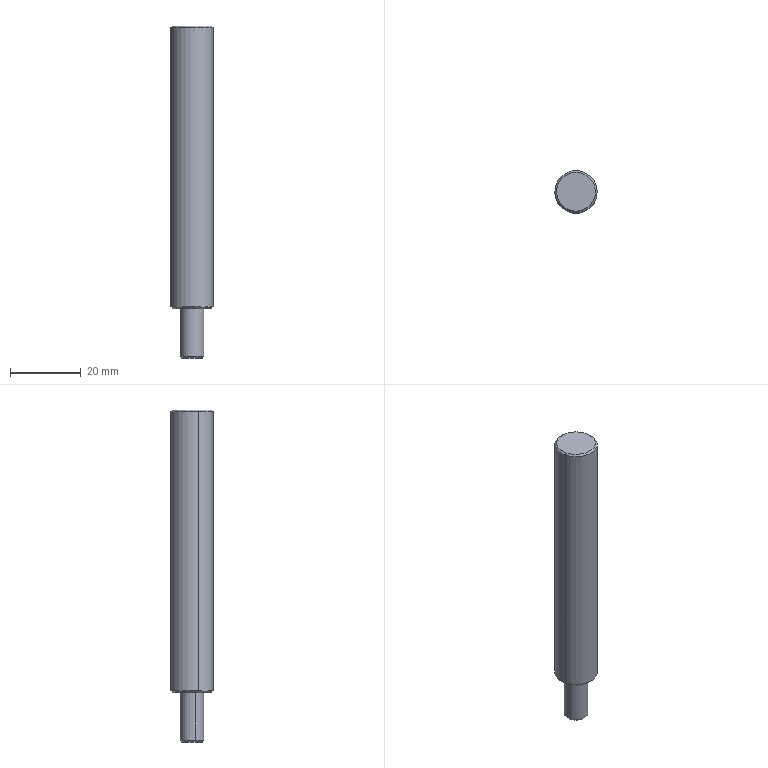Component | SolidWorks | GuidePost-2 | 1 solid | 13 faces | box 12 x 12 x 94 mm | volume 9545 mm3 | cone 6 | cylinder 4 | plane 3 | commonest cylinder face diameters 6.8 x2 12 x2
build123d program:
from build123d import *


with BuildPart() as part:
    # Sketch1 → Revolve1 (revolve)
    with BuildSketch(Plane.XY, mode=Mode.PRIVATE) as revolve1_sk:
        Polygon((0, 5.5), (0, 0), (94, 0), (94, 2.9), (93.5, 3.4), (80, 3.4), (80, 5.5), (79.5, 6), (0.5, 6), align=None)
    revolve(revolve1_sk.sketch.rotate(Axis((0, 0, 0), (1, 0, 0)), 270), axis=Axis((0, 0, 0), (1, 0, 0)))


solid = part.part

# Placed as in the assembly
solid = solid.moved(Location((0, -65, 350.554), (0, 90, 0)))
STEP:
#1=COLOUR_RGB('',0.7922,0.8196,0.9333);
#2=FILL_AREA_STYLE_COLOUR('',#1);
#3=FILL_AREA_STYLE('',(#2));
#4=SURFACE_STYLE_FILL_AREA(#3);
#5=SURFACE_SIDE_STYLE('',(#4));
#6=SURFACE_STYLE_USAGE(.BOTH.,#5);
#7=PRESENTATION_STYLE_ASSIGNMENT((#6));
#8=CARTESIAN_POINT('',(-0.109,-2.593,10.101));
#9=VERTEX_POINT('',#8);
#10=CARTESIAN_POINT('',(0.109,-2.525,10.101));
#11=VERTEX_POINT('',#10);
#12=CARTESIAN_POINT('',(-0.,-2.559,10.101));
#13=DIRECTION('',(0.,0.,-1.));
#14=DIRECTION('',(-0.9544,-0.2985,0.));
#15=AXIS2_PLACEMENT_3D('',#12,#13,#14);
#16=CIRCLE('',#15,0.1142);
#17=EDGE_CURVE('',#9,#11,#16,.T.);
#18=ORIENTED_EDGE('',*,*,#17,.F.);
#19=CARTESIAN_POINT('',(-0.1278,-2.599,10.12));
#20=VERTEX_POINT('',#19);
#21=CARTESIAN_POINT('',(-0.109,-2.593,10.101));
#22=DIRECTION('',(-0.6749,-0.2111,0.7071));
#23=VECTOR('',#22,39.37);
#24=LINE('',#21,#23);
#25=EDGE_CURVE('',#9,#20,#24,.T.);
#26=ORIENTED_EDGE('',*,*,#25,.T.);
#27=CARTESIAN_POINT('',(0.1278,-2.519,10.12));
#28=VERTEX_POINT('',#27);
#29=CARTESIAN_POINT('',(-0.,-2.559,10.12));
#30=DIRECTION('',(0.,0.,-1.));
#31=DIRECTION('',(-0.9544,-0.2985,0.));
#32=AXIS2_PLACEMENT_3D('',#29,#30,#31);
#33=CIRCLE('',#32,0.1339);
#34=EDGE_CURVE('',#20,#28,#33,.T.);
#35=ORIENTED_EDGE('',*,*,#34,.T.);
#36=CARTESIAN_POINT('',(0.109,-2.525,10.101));
#37=DIRECTION('',(0.6749,0.2111,0.7071));
#38=VECTOR('',#37,39.37);
#39=LINE('',#36,#38);
#40=EDGE_CURVE('',#11,#28,#39,.T.);
#41=ORIENTED_EDGE('',*,*,#40,.F.);
#42=EDGE_LOOP('',(#18,#26,#35,#41));
#43=FACE_OUTER_BOUND('',#42,.T.);
#44=CARTESIAN_POINT('',(-0.,-2.559,10.101));
#45=DIRECTION('',(-0.,-0.,1.));
#46=DIRECTION('',(0.9544,0.2985,0.));
#47=AXIS2_PLACEMENT_3D('',#44,#45,#46);
#48=CONICAL_SURFACE('',#47,0.1142,0.7854);
#49=ADVANCED_FACE('',(#43),#48,.T.);
#50=CARTESIAN_POINT('',(-0.1278,-2.599,10.652));
#51=VERTEX_POINT('',#50);
#52=CARTESIAN_POINT('',(0.1278,-2.519,10.652));
#53=VERTEX_POINT('',#52);
#54=CARTESIAN_POINT('',(-0.,-2.559,10.652));
#55=DIRECTION('',(0.,0.,-1.));
#56=DIRECTION('',(-0.9544,-0.2985,0.));
#57=AXIS2_PLACEMENT_3D('',#54,#55,#56);
#58=CIRCLE('',#57,0.1339);
#59=EDGE_CURVE('',#51,#53,#58,.T.);
#60=ORIENTED_EDGE('',*,*,#59,.T.);
#61=CARTESIAN_POINT('',(0.1278,-2.519,13.801));
#62=DIRECTION('',(0.,0.,-1.));
#63=VECTOR('',#62,39.37);
#64=LINE('',#61,#63);
#65=EDGE_CURVE('',#53,#28,#64,.T.);
#66=ORIENTED_EDGE('',*,*,#65,.T.);
#67=ORIENTED_EDGE('',*,*,#34,.F.);
#68=CARTESIAN_POINT('',(-0.1278,-2.599,13.801));
#69=DIRECTION('',(0.,0.,-1.));
#70=VECTOR('',#69,39.37);
#71=LINE('',#68,#70);
#72=EDGE_CURVE('',#51,#20,#71,.T.);
#73=ORIENTED_EDGE('',*,*,#72,.F.);
#74=EDGE_LOOP('',(#60,#66,#67,#73));
#75=FACE_OUTER_BOUND('',#74,.T.);
#76=CARTESIAN_POINT('',(-0.,-2.559,13.801));
#77=DIRECTION('',(0.,0.,-1.));
#78=DIRECTION('',(-0.9544,-0.2985,0.));
#79=AXIS2_PLACEMENT_3D('',#76,#77,#78);
#80=CYLINDRICAL_SURFACE('',#79,0.1339);
#81=ADVANCED_FACE('',(#75),#80,.T.);
#82=CARTESIAN_POINT('',(-0.2067,-2.624,10.652));
#83=VERTEX_POINT('',#82);
#84=CARTESIAN_POINT('',(0.2067,-2.494,10.652));
#85=VERTEX_POINT('',#84);
#86=CARTESIAN_POINT('',(-0.,-2.559,10.652));
#87=DIRECTION('',(0.,0.,-1.));
#88=DIRECTION('',(-0.9544,-0.2985,0.));
#89=AXIS2_PLACEMENT_3D('',#86,#87,#88);
#90=CIRCLE('',#89,0.2165);
#91=EDGE_CURVE('',#83,#85,#90,.T.);
#92=ORIENTED_EDGE('',*,*,#91,.F.);
#93=CARTESIAN_POINT('',(-0.2255,-2.63,10.671));
#94=VERTEX_POINT('',#93);
#95=CARTESIAN_POINT('',(-0.2067,-2.624,10.652));
#96=DIRECTION('',(-0.6749,-0.2111,0.7071));
#97=VECTOR('',#96,39.37);
#98=LINE('',#95,#97);
#99=EDGE_CURVE('',#83,#94,#98,.T.);
#100=ORIENTED_EDGE('',*,*,#99,.T.);
#101=CARTESIAN_POINT('',(0.2255,-2.489,10.671));
#102=VERTEX_POINT('',#101);
#103=CARTESIAN_POINT('',(-0.,-2.559,10.671));
#104=DIRECTION('',(0.,0.,-1.));
#105=DIRECTION('',(-0.9544,-0.2985,0.));
#106=AXIS2_PLACEMENT_3D('',#103,#104,#105);
#107=CIRCLE('',#106,0.2362);
#108=EDGE_CURVE('',#94,#102,#107,.T.);
#109=ORIENTED_EDGE('',*,*,#108,.T.);
#110=CARTESIAN_POINT('',(0.2067,-2.494,10.652));
#111=DIRECTION('',(0.6749,0.2111,0.7071));
#112=VECTOR('',#111,39.37);
#113=LINE('',#110,#112);
#114=EDGE_CURVE('',#85,#102,#113,.T.);
#115=ORIENTED_EDGE('',*,*,#114,.F.);
#116=EDGE_LOOP('',(#92,#100,#109,#115));
#117=FACE_OUTER_BOUND('',#116,.T.);
#118=CARTESIAN_POINT('',(-0.,-2.559,10.652));
#119=DIRECTION('',(-0.,-0.,1.));
#120=DIRECTION('',(0.9544,0.2985,0.));
#121=AXIS2_PLACEMENT_3D('',#118,#119,#120);
#122=CONICAL_SURFACE('',#121,0.2165,0.7854);
#123=ADVANCED_FACE('',(#117),#122,.T.);
#124=CARTESIAN_POINT('',(-0.2255,-2.63,13.782));
#125=VERTEX_POINT('',#124);
#126=CARTESIAN_POINT('',(0.2255,-2.489,13.782));
#127=VERTEX_POINT('',#126);
#128=CARTESIAN_POINT('',(-0.,-2.559,13.782));
#129=DIRECTION('',(0.,0.,-1.));
#130=DIRECTION('',(-0.9544,-0.2985,0.));
#131=AXIS2_PLACEMENT_3D('',#128,#129,#130);
#132=CIRCLE('',#131,0.2362);
#133=EDGE_CURVE('',#125,#127,#132,.T.);
#134=ORIENTED_EDGE('',*,*,#133,.T.);
#135=CARTESIAN_POINT('',(0.2255,-2.489,13.801));
#136=DIRECTION('',(0.,0.,-1.));
#137=VECTOR('',#136,39.37);
#138=LINE('',#135,#137);
#139=EDGE_CURVE('',#127,#102,#138,.T.);
#140=ORIENTED_EDGE('',*,*,#139,.T.);
#141=ORIENTED_EDGE('',*,*,#108,.F.);
#142=CARTESIAN_POINT('',(-0.2255,-2.63,13.801));
#143=DIRECTION('',(0.,0.,-1.));
#144=VECTOR('',#143,39.37);
#145=LINE('',#142,#144);
#146=EDGE_CURVE('',#125,#94,#145,.T.);
#147=ORIENTED_EDGE('',*,*,#146,.F.);
#148=EDGE_LOOP('',(#134,#140,#141,#147));
#149=FACE_OUTER_BOUND('',#148,.T.);
#150=CARTESIAN_POINT('',(-0.,-2.559,13.801));
#151=DIRECTION('',(0.,0.,-1.));
#152=DIRECTION('',(-0.9544,-0.2985,0.));
#153=AXIS2_PLACEMENT_3D('',#150,#151,#152);
#154=CYLINDRICAL_SURFACE('',#153,0.2362);
#155=ADVANCED_FACE('',(#149),#154,.T.);
#156=CARTESIAN_POINT('',(-0.2067,-2.624,13.801));
#157=VERTEX_POINT('',#156);
#158=CARTESIAN_POINT('',(0.2067,-2.494,13.801));
#159=VERTEX_POINT('',#158);
#160=CARTESIAN_POINT('',(-0.,-2.559,13.801));
#161=DIRECTION('',(0.,0.,-1.));
#162=DIRECTION('',(-0.9544,-0.2985,0.));
#163=AXIS2_PLACEMENT_3D('',#160,#161,#162);
#164=CIRCLE('',#163,0.2165);
#165=EDGE_CURVE('',#157,#159,#164,.T.);
#166=ORIENTED_EDGE('',*,*,#165,.T.);
#167=CARTESIAN_POINT('',(0.2255,-2.489,13.782));
#168=DIRECTION('',(0.6749,0.2111,-0.7071));
#169=VECTOR('',#168,39.37);
#170=LINE('',#167,#169);
#171=EDGE_CURVE('',#159,#127,#170,.T.);
#172=ORIENTED_EDGE('',*,*,#171,.T.);
#173=ORIENTED_EDGE('',*,*,#133,.F.);
#174=CARTESIAN_POINT('',(-0.2255,-2.63,13.782));
#175=DIRECTION('',(-0.6749,-0.2111,-0.7071));
#176=VECTOR('',#175,39.37);
#177=LINE('',#174,#176);
#178=EDGE_CURVE('',#157,#125,#177,.T.);
#179=ORIENTED_EDGE('',*,*,#178,.F.);
#180=EDGE_LOOP('',(#166,#172,#173,#179));
#181=FACE_OUTER_BOUND('',#180,.T.);
#182=CARTESIAN_POINT('',(-0.,-2.559,13.782));
#183=DIRECTION('',(0.,0.,-1.));
#184=DIRECTION('',(-0.9544,-0.2985,0.));
#185=AXIS2_PLACEMENT_3D('',#182,#183,#184);
#186=CONICAL_SURFACE('',#185,0.2362,0.7854);
#187=ADVANCED_FACE('',(#181),#186,.T.);
#188=ORIENTED_EDGE('',*,*,#171,.F.);
#189=CARTESIAN_POINT('',(-0.,-2.559,13.801));
#190=DIRECTION('',(0.,0.,-1.));
#191=DIRECTION('',(-0.9544,-0.2985,0.));
#192=AXIS2_PLACEMENT_3D('',#189,#190,#191);
#193=CIRCLE('',#192,0.2165);
#194=EDGE_CURVE('',#159,#157,#193,.T.);
#195=ORIENTED_EDGE('',*,*,#194,.T.);
#196=ORIENTED_EDGE('',*,*,#178,.T.);
#197=CARTESIAN_POINT('',(-0.,-2.559,13.782));
#198=DIRECTION('',(0.,0.,-1.));
#199=DIRECTION('',(-0.9544,-0.2985,0.));
#200=AXIS2_PLACEMENT_3D('',#197,#198,#199);
#201=CIRCLE('',#200,0.2362);
#202=EDGE_CURVE('',#127,#125,#201,.T.);
#203=ORIENTED_EDGE('',*,*,#202,.F.);
#204=EDGE_LOOP('',(#188,#195,#196,#203));
#205=FACE_OUTER_BOUND('',#204,.T.);
#206=CARTESIAN_POINT('',(-0.,-2.559,13.782));
#207=DIRECTION('',(0.,0.,-1.));
#208=DIRECTION('',(-0.9544,-0.2985,0.));
#209=AXIS2_PLACEMENT_3D('',#206,#207,#208);
#210=CONICAL_SURFACE('',#209,0.2362,0.7854);
#211=ADVANCED_FACE('',(#205),#210,.T.);
#212=ORIENTED_EDGE('',*,*,#139,.F.);
#213=ORIENTED_EDGE('',*,*,#202,.T.);
#214=ORIENTED_EDGE('',*,*,#146,.T.);
#215=CARTESIAN_POINT('',(-0.,-2.559,10.671));
#216=DIRECTION('',(0.,0.,-1.));
#217=DIRECTION('',(-0.9544,-0.2985,0.));
#218=AXIS2_PLACEMENT_3D('',#215,#216,#217);
#219=CIRCLE('',#218,0.2362);
#220=EDGE_CURVE('',#102,#94,#219,.T.);
#221=ORIENTED_EDGE('',*,*,#220,.F.);
#222=EDGE_LOOP('',(#212,#213,#214,#221));
#223=FACE_OUTER_BOUND('',#222,.T.);
#224=CARTESIAN_POINT('',(-0.,-2.559,13.801));
#225=DIRECTION('',(0.,0.,-1.));
#226=DIRECTION('',(-0.9544,-0.2985,0.));
#227=AXIS2_PLACEMENT_3D('',#224,#225,#226);
#228=CYLINDRICAL_SURFACE('',#227,0.2362);
#229=ADVANCED_FACE('',(#223),#228,.T.);
#230=ORIENTED_EDGE('',*,*,#99,.F.);
#231=CARTESIAN_POINT('',(-0.,-2.559,10.652));
#232=DIRECTION('',(0.,0.,-1.));
#233=DIRECTION('',(-0.9544,-0.2985,0.));
#234=AXIS2_PLACEMENT_3D('',#231,#232,#233);
#235=CIRCLE('',#234,0.2165);
#236=EDGE_CURVE('',#85,#83,#235,.T.);
#237=ORIENTED_EDGE('',*,*,#236,.F.);
#238=ORIENTED_EDGE('',*,*,#114,.T.);
#239=ORIENTED_EDGE('',*,*,#220,.T.);
#240=EDGE_LOOP('',(#230,#237,#238,#239));
#241=FACE_OUTER_BOUND('',#240,.T.);
#242=CARTESIAN_POINT('',(-0.,-2.559,10.652));
#243=DIRECTION('',(-0.,-0.,1.));
#244=DIRECTION('',(0.9544,0.2985,0.));
#245=AXIS2_PLACEMENT_3D('',#242,#243,#244);
#246=CONICAL_SURFACE('',#245,0.2165,0.7854);
#247=ADVANCED_FACE('',(#241),#246,.T.);
#248=ORIENTED_EDGE('',*,*,#236,.T.);
#249=ORIENTED_EDGE('',*,*,#91,.T.);
#250=EDGE_LOOP('',(#248,#249));
#251=FACE_OUTER_BOUND('',#250,.T.);
#252=ORIENTED_EDGE('',*,*,#59,.F.);
#253=CARTESIAN_POINT('',(-0.,-2.559,10.652));
#254=DIRECTION('',(0.,0.,-1.));
#255=DIRECTION('',(-0.9544,-0.2985,0.));
#256=AXIS2_PLACEMENT_3D('',#253,#254,#255);
#257=CIRCLE('',#256,0.1339);
#258=EDGE_CURVE('',#53,#51,#257,.T.);
#259=ORIENTED_EDGE('',*,*,#258,.F.);
#260=EDGE_LOOP('',(#252,#259));
#261=FACE_BOUND('',#260,.T.);
#262=CARTESIAN_POINT('',(-0.03995,-2.431,10.652));
#263=DIRECTION('',(0.,0.,-1.));
#264=DIRECTION('',(-0.9544,-0.2985,-0.));
#265=AXIS2_PLACEMENT_3D('',#262,#263,#264);
#266=PLANE('',#265);
#267=ADVANCED_FACE('',(#251,#261),#266,.T.);
#268=ORIENTED_EDGE('',*,*,#65,.F.);
#269=ORIENTED_EDGE('',*,*,#258,.T.);
#270=ORIENTED_EDGE('',*,*,#72,.T.);
#271=CARTESIAN_POINT('',(-0.,-2.559,10.12));
#272=DIRECTION('',(0.,0.,-1.));
#273=DIRECTION('',(-0.9544,-0.2985,0.));
#274=AXIS2_PLACEMENT_3D('',#271,#272,#273);
#275=CIRCLE('',#274,0.1339);
#276=EDGE_CURVE('',#28,#20,#275,.T.);
#277=ORIENTED_EDGE('',*,*,#276,.F.);
#278=EDGE_LOOP('',(#268,#269,#270,#277));
#279=FACE_OUTER_BOUND('',#278,.T.);
#280=CARTESIAN_POINT('',(-0.,-2.559,13.801));
#281=DIRECTION('',(0.,0.,-1.));
#282=DIRECTION('',(-0.9544,-0.2985,0.));
#283=AXIS2_PLACEMENT_3D('',#280,#281,#282);
#284=CYLINDRICAL_SURFACE('',#283,0.1339);
#285=ADVANCED_FACE('',(#279),#284,.T.);
#286=ORIENTED_EDGE('',*,*,#25,.F.);
#287=CARTESIAN_POINT('',(-0.,-2.559,10.101));
#288=DIRECTION('',(0.,0.,-1.));
#289=DIRECTION('',(-0.9544,-0.2985,0.));
#290=AXIS2_PLACEMENT_3D('',#287,#288,#289);
#291=CIRCLE('',#290,0.1142);
#292=EDGE_CURVE('',#11,#9,#291,.T.);
#293=ORIENTED_EDGE('',*,*,#292,.F.);
#294=ORIENTED_EDGE('',*,*,#40,.T.);
#295=ORIENTED_EDGE('',*,*,#276,.T.);
#296=EDGE_LOOP('',(#286,#293,#294,#295));
#297=FACE_OUTER_BOUND('',#296,.T.);
#298=CARTESIAN_POINT('',(-0.,-2.559,10.101));
#299=DIRECTION('',(-0.,-0.,1.));
#300=DIRECTION('',(0.9544,0.2985,0.));
#301=AXIS2_PLACEMENT_3D('',#298,#299,#300);
#302=CONICAL_SURFACE('',#301,0.1142,0.7854);
#303=ADVANCED_FACE('',(#297),#302,.T.);
#304=ORIENTED_EDGE('',*,*,#292,.T.);
#305=ORIENTED_EDGE('',*,*,#17,.T.);
#306=EDGE_LOOP('',(#304,#305));
#307=FACE_OUTER_BOUND('',#306,.T.);
#308=CARTESIAN_POINT('',(-0.,-2.559,10.101));
#309=DIRECTION('',(0.,0.,-1.));
#310=DIRECTION('',(-0.9544,-0.2985,-0.));
#311=AXIS2_PLACEMENT_3D('',#308,#309,#310);
#312=PLANE('',#311);
#313=ADVANCED_FACE('',(#307),#312,.T.);
#314=ORIENTED_EDGE('',*,*,#165,.F.);
#315=ORIENTED_EDGE('',*,*,#194,.F.);
#316=EDGE_LOOP('',(#314,#315));
#317=FACE_OUTER_BOUND('',#316,.T.);
#318=CARTESIAN_POINT('',(-0.06463,-2.352,13.801));
#319=DIRECTION('',(-0.,-0.,1.));
#320=DIRECTION('',(0.9544,0.2985,0.));
#321=AXIS2_PLACEMENT_3D('',#318,#319,#320);
#322=PLANE('',#321);
#323=ADVANCED_FACE('',(#317),#322,.T.);
#324=CLOSED_SHELL('',(#49,#81,#123,#155,#187,#211,#229,#247,#267,#285,#303,#313,#323));
#325=MANIFOLD_SOLID_BREP('',#324);
#326=STYLED_ITEM('',(#7),#325);
#327=(LENGTH_UNIT()NAMED_UNIT(*)SI_UNIT($,.METRE.));
#328=LENGTH_MEASURE_WITH_UNIT(LENGTH_MEASURE(0.0254),#327);
#329=DIMENSIONAL_EXPONENTS(1.,0.,0.,0.,0.,0.,0.);
#330=(CONVERSION_BASED_UNIT('',#328)LENGTH_UNIT()NAMED_UNIT(#329));
#331=UNCERTAINTY_MEASURE_WITH_UNIT(LENGTH_MEASURE(0.00001),#330,'','');
#332=(NAMED_UNIT(*)PLANE_ANGLE_UNIT()SI_UNIT($,.RADIAN.));
#333=(NAMED_UNIT(*)SI_UNIT($,.STERADIAN.)SOLID_ANGLE_UNIT());
#334=(GEOMETRIC_REPRESENTATION_CONTEXT(3)GLOBAL_UNCERTAINTY_ASSIGNED_CONTEXT((#331))GLOBAL_UNIT_ASSIGNED_CONTEXT((#330,#332,#333))REPRESENTATION_CONTEXT('',''));
#335=MECHANICAL_DESIGN_GEOMETRIC_PRESENTATION_REPRESENTATION('',(#326),#334);
#336=CARTESIAN_POINT('',(0.,0.,0.));
#337=DIRECTION('',(0.,0.,1.));
#338=DIRECTION('',(1.,0.,0.));
#339=AXIS2_PLACEMENT_3D('',#336,#337,#338);
#340=(LENGTH_UNIT()NAMED_UNIT(*)SI_UNIT($,.METRE.));
#341=LENGTH_MEASURE_WITH_UNIT(LENGTH_MEASURE(0.0254),#340);
#342=DIMENSIONAL_EXPONENTS(1.,0.,0.,0.,0.,0.,0.);
#343=(CONVERSION_BASED_UNIT('',#341)LENGTH_UNIT()NAMED_UNIT(#342));
#344=UNCERTAINTY_MEASURE_WITH_UNIT(LENGTH_MEASURE(0.00001),#343,'','');
#345=(NAMED_UNIT(*)PLANE_ANGLE_UNIT()SI_UNIT($,.RADIAN.));
#346=(NAMED_UNIT(*)SI_UNIT($,.STERADIAN.)SOLID_ANGLE_UNIT());
#347=(GEOMETRIC_REPRESENTATION_CONTEXT(3)GLOBAL_UNCERTAINTY_ASSIGNED_CONTEXT((#344))GLOBAL_UNIT_ASSIGNED_CONTEXT((#343,#345,#346))REPRESENTATION_CONTEXT('',''));
#348=ADVANCED_BREP_SHAPE_REPRESENTATION('',(#325,#339),#347);
#349=PRESENTATION_LAYER_ASSIGNMENT('','',(#326));